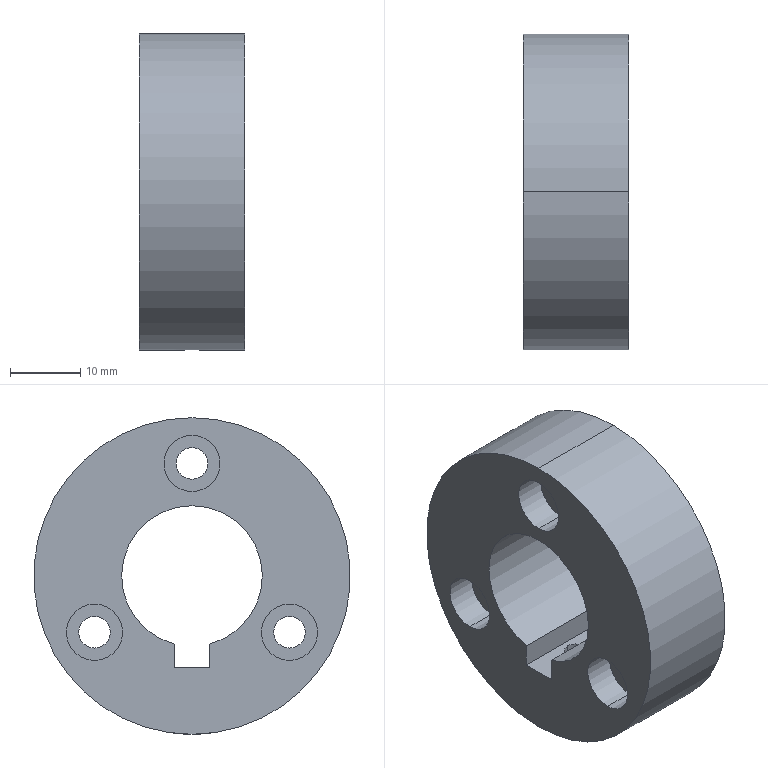Component | SolidWorks | 18-1 | 1 solid | 26 faces | box 15 x 45 x 45 mm | volume 17661 mm3 | cylinder 18 | plane 8 | commonest cylinder face diameters 8 x6 4.5 x6 3.3 x2 20 x2 45 x2
build123d program:
from build123d import *

# Parameters (mm, degrees)
SKETCH1_R                                       = 22.5
SKETCH1_R_2                                     = 10
EXTRUDE1_DEPTH                                  = 15
SKETCH2_W                                       = 5
SKETCH2_H                                       = 5
EXTRUDE2_DEPTH                                  = 36.178
M4_HEX_SOCKET_HEAD_CAP_SCREW_CBORE1_D           = 4.5
M4_HEX_SOCKET_HEAD_CAP_SCREW_CBORE1_CBORE_D     = 8
M4_HEX_SOCKET_HEAD_CAP_SCREW_CBORE1_CBORE_DEPTH = 4.4
M4_TAPPED_HOLE1_D                               = 3.3
M4_TAPPED_HOLE1_DEPTH                           = 9.5


with BuildPart() as part:
    # Sketch1 → Extrude1 (new body)
    with BuildSketch(Plane(origin=(0, 0, 0), x_dir=(1, 0, 0), z_dir=(0, 1, 0))):
        with Locations(Location((0, 0, 0), (0, 0, 270))):
            Circle(SKETCH1_R)
        with Locations(Location((0, 0, 0), (0, 0, 270))):
            Circle(SKETCH1_R_2, mode=Mode.SUBTRACT)
    extrude(amount=EXTRUDE1_DEPTH)

    # Sketch2 → Extrude2 (cut, through all)
    with BuildSketch(Plane(origin=(0, 15, 0), x_dir=(1, 0, 0), z_dir=(0, 1, 0))):
        with Locations((0, -10.5)):
            Rectangle(SKETCH2_W, SKETCH2_H)
    extrude(amount=-EXTRUDE2_DEPTH, mode=Mode.SUBTRACT)

    # M4 Hex Socket Head Cap Screw CBORE1 (through all)
    with Locations(Plane(origin=(13.856, 0, 8), x_dir=(0, 0, -1), z_dir=(0, -1, 0))):
        with Locations((0, 0), (0, -27.713), (24, -13.856)):
            CounterBoreHole(M4_HEX_SOCKET_HEAD_CAP_SCREW_CBORE1_D / 2, M4_HEX_SOCKET_HEAD_CAP_SCREW_CBORE1_CBORE_D / 2, M4_HEX_SOCKET_HEAD_CAP_SCREW_CBORE1_CBORE_DEPTH)

    # M4 Tapped Hole1
    with Locations(Plane(origin=(0, 0, 13), x_dir=(-1, 0, 0), z_dir=(0, 0, -1))):
        with Locations((0, 7.5)):
            Hole(M4_TAPPED_HOLE1_D / 2, depth=M4_TAPPED_HOLE1_DEPTH)


solid = part.part

# Placed as in the assembly
solid = solid.moved(Location((63.5, -32.5, 30), (180, 0, -90)))
STEP:
#1=CARTESIAN_POINT('',(2.795,-1.215,0.2977));
#2=VERTEX_POINT('',#1);
#3=CARTESIAN_POINT('',(2.73,-1.28,0.2953));
#4=VERTEX_POINT('',#3);
#5=CARTESIAN_POINT('',(2.795,-1.215,0.2977));
#6=CARTESIAN_POINT('',(2.787,-1.215,0.2977));
#7=CARTESIAN_POINT('',(2.778,-1.216,0.2975));
#8=CARTESIAN_POINT('',(2.766,-1.221,0.2972));
#9=CARTESIAN_POINT('',(2.763,-1.223,0.2971));
#10=CARTESIAN_POINT('',(2.756,-1.228,0.2968));
#11=CARTESIAN_POINT('',(2.752,-1.231,0.2966));
#12=CARTESIAN_POINT('',(2.743,-1.24,0.2962));
#13=CARTESIAN_POINT('',(2.739,-1.247,0.2958));
#14=CARTESIAN_POINT('',(2.732,-1.262,0.2954));
#15=CARTESIAN_POINT('',(2.73,-1.271,0.2953));
#16=CARTESIAN_POINT('',(2.73,-1.28,0.2953));
#17=B_SPLINE_CURVE_WITH_KNOTS('',3,(#5,#6,#7,#8,#9,#10,#11,#12,#13,#14,#15,#16),.UNSPECIFIED.,.F.,.F.,(4,2,2,2,2,4),(0.007741,0.008386,0.008708,0.00903,0.009675,0.01032),.UNSPECIFIED.);
#18=EDGE_CURVE('',#2,#4,#17,.T.);
#19=ORIENTED_EDGE('',*,*,#18,.F.);
#20=CARTESIAN_POINT('',(2.795,-1.215,0.6693));
#21=VERTEX_POINT('',#20);
#22=CARTESIAN_POINT('',(2.795,-1.215,0.6693));
#23=DIRECTION('',(0.,0.,1.));
#24=VECTOR('',#23,39.37);
#25=LINE('',#22,#24);
#26=EDGE_CURVE('',#2,#21,#25,.T.);
#27=ORIENTED_EDGE('',*,*,#26,.T.);
#28=CARTESIAN_POINT('',(2.795,-1.344,0.6693));
#29=VERTEX_POINT('',#28);
#30=CARTESIAN_POINT('',(2.795,-1.28,0.6693));
#31=DIRECTION('',(0.,0.,1.));
#32=DIRECTION('',(0.,-1.,0.));
#33=AXIS2_PLACEMENT_3D('',#30,#31,#32);
#34=CIRCLE('',#33,0.06496);
#35=EDGE_CURVE('',#21,#29,#34,.T.);
#36=ORIENTED_EDGE('',*,*,#35,.T.);
#37=CARTESIAN_POINT('',(2.795,-1.344,0.2977));
#38=VERTEX_POINT('',#37);
#39=CARTESIAN_POINT('',(2.795,-1.344,0.6693));
#40=DIRECTION('',(0.,0.,1.));
#41=VECTOR('',#40,39.37);
#42=LINE('',#39,#41);
#43=EDGE_CURVE('',#38,#29,#42,.T.);
#44=ORIENTED_EDGE('',*,*,#43,.F.);
#45=CARTESIAN_POINT('',(2.73,-1.28,0.2953));
#46=CARTESIAN_POINT('',(2.73,-1.284,0.2953));
#47=CARTESIAN_POINT('',(2.731,-1.288,0.2953));
#48=CARTESIAN_POINT('',(2.732,-1.296,0.2954));
#49=CARTESIAN_POINT('',(2.734,-1.3,0.2955));
#50=CARTESIAN_POINT('',(2.737,-1.308,0.2957));
#51=CARTESIAN_POINT('',(2.739,-1.312,0.2959));
#52=CARTESIAN_POINT('',(2.744,-1.319,0.2962));
#53=CARTESIAN_POINT('',(2.746,-1.322,0.2963));
#54=CARTESIAN_POINT('',(2.755,-1.331,0.2968));
#55=CARTESIAN_POINT('',(2.763,-1.336,0.2971));
#56=CARTESIAN_POINT('',(2.778,-1.343,0.2975));
#57=CARTESIAN_POINT('',(2.787,-1.344,0.2977));
#58=CARTESIAN_POINT('',(2.795,-1.344,0.2977));
#59=B_SPLINE_CURVE_WITH_KNOTS('',3,(#45,#46,#47,#48,#49,#50,#51,#52,#53,#54,#55,#56,#57,#58),.UNSPECIFIED.,.F.,.F.,(4,2,2,2,2,2,4),(0.,0.0003226,0.0006452,0.0009678,0.00129,0.001936,0.002581),.UNSPECIFIED.);
#60=EDGE_CURVE('',#4,#38,#59,.T.);
#61=ORIENTED_EDGE('',*,*,#60,.F.);
#62=EDGE_LOOP('',(#19,#27,#36,#44,#61));
#63=FACE_OUTER_BOUND('',#62,.T.);
#64=CARTESIAN_POINT('',(2.795,-1.28,0.6693));
#65=DIRECTION('',(0.,0.,1.));
#66=DIRECTION('',(0.,-1.,0.));
#67=AXIS2_PLACEMENT_3D('',#64,#65,#66);
#68=CYLINDRICAL_SURFACE('',#67,0.06496);
#69=ADVANCED_FACE('',(#63),#68,.F.);
#70=CARTESIAN_POINT('',(2.673,-0.734,0.7087));
#71=VERTEX_POINT('',#70);
#72=CARTESIAN_POINT('',(2.673,-0.734,1.024));
#73=VERTEX_POINT('',#72);
#74=CARTESIAN_POINT('',(2.673,-0.734,0.8661));
#75=DIRECTION('',(-1.,-0.,0.));
#76=DIRECTION('',(0.,0.,1.));
#77=AXIS2_PLACEMENT_3D('',#74,#75,#76);
#78=CIRCLE('',#77,0.1575);
#79=EDGE_CURVE('',#71,#73,#78,.T.);
#80=ORIENTED_EDGE('',*,*,#79,.F.);
#81=CARTESIAN_POINT('',(2.5,-0.734,0.7087));
#82=VERTEX_POINT('',#81);
#83=CARTESIAN_POINT('',(2.5,-0.734,0.7087));
#84=DIRECTION('',(-1.,-0.,0.));
#85=VECTOR('',#84,39.37);
#86=LINE('',#83,#85);
#87=EDGE_CURVE('',#71,#82,#86,.T.);
#88=ORIENTED_EDGE('',*,*,#87,.T.);
#89=CARTESIAN_POINT('',(2.5,-0.734,1.024));
#90=VERTEX_POINT('',#89);
#91=CARTESIAN_POINT('',(2.5,-0.734,0.8661));
#92=DIRECTION('',(-1.,-0.,0.));
#93=DIRECTION('',(0.,0.,1.));
#94=AXIS2_PLACEMENT_3D('',#91,#92,#93);
#95=CIRCLE('',#94,0.1575);
#96=EDGE_CURVE('',#82,#90,#95,.T.);
#97=ORIENTED_EDGE('',*,*,#96,.T.);
#98=CARTESIAN_POINT('',(2.5,-0.734,1.024));
#99=DIRECTION('',(-1.,-0.,0.));
#100=VECTOR('',#99,39.37);
#101=LINE('',#98,#100);
#102=EDGE_CURVE('',#73,#90,#101,.T.);
#103=ORIENTED_EDGE('',*,*,#102,.F.);
#104=EDGE_LOOP('',(#80,#88,#97,#103));
#105=FACE_OUTER_BOUND('',#104,.T.);
#106=CARTESIAN_POINT('',(2.5,-0.734,0.8661));
#107=DIRECTION('',(-1.,-0.,0.));
#108=DIRECTION('',(0.,0.,1.));
#109=AXIS2_PLACEMENT_3D('',#106,#107,#108);
#110=CYLINDRICAL_SURFACE('',#109,0.1575);
#111=ADVANCED_FACE('',(#105),#110,.F.);
#112=CARTESIAN_POINT('',(3.091,-0.734,0.7776));
#113=VERTEX_POINT('',#112);
#114=CARTESIAN_POINT('',(3.091,-0.734,0.9547));
#115=VERTEX_POINT('',#114);
#116=CARTESIAN_POINT('',(3.091,-0.734,0.8661));
#117=DIRECTION('',(-1.,-0.,0.));
#118=DIRECTION('',(0.,0.,1.));
#119=AXIS2_PLACEMENT_3D('',#116,#117,#118);
#120=CIRCLE('',#119,0.08858);
#121=EDGE_CURVE('',#113,#115,#120,.T.);
#122=ORIENTED_EDGE('',*,*,#121,.F.);
#123=CARTESIAN_POINT('',(2.673,-0.734,0.7776));
#124=VERTEX_POINT('',#123);
#125=CARTESIAN_POINT('',(2.5,-0.734,0.7776));
#126=DIRECTION('',(-1.,-0.,0.));
#127=VECTOR('',#126,39.37);
#128=LINE('',#125,#127);
#129=EDGE_CURVE('',#113,#124,#128,.T.);
#130=ORIENTED_EDGE('',*,*,#129,.T.);
#131=CARTESIAN_POINT('',(2.673,-0.734,0.9547));
#132=VERTEX_POINT('',#131);
#133=CARTESIAN_POINT('',(2.673,-0.734,0.8661));
#134=DIRECTION('',(-1.,-0.,0.));
#135=DIRECTION('',(0.,0.,1.));
#136=AXIS2_PLACEMENT_3D('',#133,#134,#135);
#137=CIRCLE('',#136,0.08858);
#138=EDGE_CURVE('',#124,#132,#137,.T.);
#139=ORIENTED_EDGE('',*,*,#138,.T.);
#140=CARTESIAN_POINT('',(2.5,-0.734,0.9547));
#141=DIRECTION('',(-1.,-0.,0.));
#142=VECTOR('',#141,39.37);
#143=LINE('',#140,#142);
#144=EDGE_CURVE('',#115,#132,#143,.T.);
#145=ORIENTED_EDGE('',*,*,#144,.F.);
#146=EDGE_LOOP('',(#122,#130,#139,#145));
#147=FACE_OUTER_BOUND('',#146,.T.);
#148=CARTESIAN_POINT('',(2.5,-0.734,0.8661));
#149=DIRECTION('',(-1.,-0.,0.));
#150=DIRECTION('',(0.,0.,1.));
#151=AXIS2_PLACEMENT_3D('',#148,#149,#150);
#152=CYLINDRICAL_SURFACE('',#151,0.08858);
#153=ADVANCED_FACE('',(#147),#152,.F.);
#154=CARTESIAN_POINT('',(2.673,-1.825,0.7087));
#155=VERTEX_POINT('',#154);
#156=CARTESIAN_POINT('',(2.673,-1.825,1.024));
#157=VERTEX_POINT('',#156);
#158=CARTESIAN_POINT('',(2.673,-1.825,0.8661));
#159=DIRECTION('',(-1.,-0.,0.));
#160=DIRECTION('',(0.,0.,1.));
#161=AXIS2_PLACEMENT_3D('',#158,#159,#160);
#162=CIRCLE('',#161,0.1575);
#163=EDGE_CURVE('',#155,#157,#162,.T.);
#164=ORIENTED_EDGE('',*,*,#163,.F.);
#165=CARTESIAN_POINT('',(2.5,-1.825,0.7087));
#166=VERTEX_POINT('',#165);
#167=CARTESIAN_POINT('',(2.5,-1.825,0.7087));
#168=DIRECTION('',(-1.,-0.,0.));
#169=VECTOR('',#168,39.37);
#170=LINE('',#167,#169);
#171=EDGE_CURVE('',#155,#166,#170,.T.);
#172=ORIENTED_EDGE('',*,*,#171,.T.);
#173=CARTESIAN_POINT('',(2.5,-1.825,1.024));
#174=VERTEX_POINT('',#173);
#175=CARTESIAN_POINT('',(2.5,-1.825,0.8661));
#176=DIRECTION('',(-1.,-0.,0.));
#177=DIRECTION('',(0.,0.,1.));
#178=AXIS2_PLACEMENT_3D('',#175,#176,#177);
#179=CIRCLE('',#178,0.1575);
#180=EDGE_CURVE('',#166,#174,#179,.T.);
#181=ORIENTED_EDGE('',*,*,#180,.T.);
#182=CARTESIAN_POINT('',(2.5,-1.825,1.024));
#183=DIRECTION('',(-1.,-0.,0.));
#184=VECTOR('',#183,39.37);
#185=LINE('',#182,#184);
#186=EDGE_CURVE('',#157,#174,#185,.T.);
#187=ORIENTED_EDGE('',*,*,#186,.F.);
#188=EDGE_LOOP('',(#164,#172,#181,#187));
#189=FACE_OUTER_BOUND('',#188,.T.);
#190=CARTESIAN_POINT('',(2.5,-1.825,0.8661));
#191=DIRECTION('',(-1.,-0.,0.));
#192=DIRECTION('',(0.,0.,1.));
#193=AXIS2_PLACEMENT_3D('',#190,#191,#192);
#194=CYLINDRICAL_SURFACE('',#193,0.1575);
#195=ADVANCED_FACE('',(#189),#194,.F.);
#196=CARTESIAN_POINT('',(3.091,-1.825,0.7776));
#197=VERTEX_POINT('',#196);
#198=CARTESIAN_POINT('',(3.091,-1.825,0.9547));
#199=VERTEX_POINT('',#198);
#200=CARTESIAN_POINT('',(3.091,-1.825,0.8661));
#201=DIRECTION('',(-1.,-0.,0.));
#202=DIRECTION('',(0.,0.,1.));
#203=AXIS2_PLACEMENT_3D('',#200,#201,#202);
#204=CIRCLE('',#203,0.08858);
#205=EDGE_CURVE('',#197,#199,#204,.T.);
#206=ORIENTED_EDGE('',*,*,#205,.F.);
#207=CARTESIAN_POINT('',(2.673,-1.825,0.7776));
#208=VERTEX_POINT('',#207);
#209=CARTESIAN_POINT('',(2.5,-1.825,0.7776));
#210=DIRECTION('',(-1.,-0.,0.));
#211=VECTOR('',#210,39.37);
#212=LINE('',#209,#211);
#213=EDGE_CURVE('',#197,#208,#212,.T.);
#214=ORIENTED_EDGE('',*,*,#213,.T.);
#215=CARTESIAN_POINT('',(2.673,-1.825,0.9547));
#216=VERTEX_POINT('',#215);
#217=CARTESIAN_POINT('',(2.673,-1.825,0.8661));
#218=DIRECTION('',(-1.,-0.,0.));
#219=DIRECTION('',(0.,0.,1.));
#220=AXIS2_PLACEMENT_3D('',#217,#218,#219);
#221=CIRCLE('',#220,0.08858);
#222=EDGE_CURVE('',#208,#216,#221,.T.);
#223=ORIENTED_EDGE('',*,*,#222,.T.);
#224=CARTESIAN_POINT('',(2.5,-1.825,0.9547));
#225=DIRECTION('',(-1.,-0.,0.));
#226=VECTOR('',#225,39.37);
#227=LINE('',#224,#226);
#228=EDGE_CURVE('',#199,#216,#227,.T.);
#229=ORIENTED_EDGE('',*,*,#228,.F.);
#230=EDGE_LOOP('',(#206,#214,#223,#229));
#231=FACE_OUTER_BOUND('',#230,.T.);
#232=CARTESIAN_POINT('',(2.5,-1.825,0.8661));
#233=DIRECTION('',(-1.,-0.,0.));
#234=DIRECTION('',(0.,0.,1.));
#235=AXIS2_PLACEMENT_3D('',#232,#233,#234);
#236=CYLINDRICAL_SURFACE('',#235,0.08858);
#237=ADVANCED_FACE('',(#231),#236,.F.);
#238=CARTESIAN_POINT('',(2.673,-1.28,1.654));
#239=VERTEX_POINT('',#238);
#240=CARTESIAN_POINT('',(2.673,-1.28,1.969));
#241=VERTEX_POINT('',#240);
#242=CARTESIAN_POINT('',(2.673,-1.28,1.811));
#243=DIRECTION('',(-1.,-0.,0.));
#244=DIRECTION('',(0.,0.,1.));
#245=AXIS2_PLACEMENT_3D('',#242,#243,#244);
#246=CIRCLE('',#245,0.1575);
#247=EDGE_CURVE('',#239,#241,#246,.T.);
#248=ORIENTED_EDGE('',*,*,#247,.F.);
#249=CARTESIAN_POINT('',(2.5,-1.28,1.654));
#250=VERTEX_POINT('',#249);
#251=CARTESIAN_POINT('',(2.5,-1.28,1.654));
#252=DIRECTION('',(-1.,-0.,0.));
#253=VECTOR('',#252,39.37);
#254=LINE('',#251,#253);
#255=EDGE_CURVE('',#239,#250,#254,.T.);
#256=ORIENTED_EDGE('',*,*,#255,.T.);
#257=CARTESIAN_POINT('',(2.5,-1.28,1.969));
#258=VERTEX_POINT('',#257);
#259=CARTESIAN_POINT('',(2.5,-1.28,1.811));
#260=DIRECTION('',(-1.,-0.,0.));
#261=DIRECTION('',(0.,0.,1.));
#262=AXIS2_PLACEMENT_3D('',#259,#260,#261);
#263=CIRCLE('',#262,0.1575);
#264=EDGE_CURVE('',#250,#258,#263,.T.);
#265=ORIENTED_EDGE('',*,*,#264,.T.);
#266=CARTESIAN_POINT('',(2.5,-1.28,1.969));
#267=DIRECTION('',(-1.,-0.,0.));
#268=VECTOR('',#267,39.37);
#269=LINE('',#266,#268);
#270=EDGE_CURVE('',#241,#258,#269,.T.);
#271=ORIENTED_EDGE('',*,*,#270,.F.);
#272=EDGE_LOOP('',(#248,#256,#265,#271));
#273=FACE_OUTER_BOUND('',#272,.T.);
#274=CARTESIAN_POINT('',(2.5,-1.28,1.811));
#275=DIRECTION('',(-1.,-0.,0.));
#276=DIRECTION('',(0.,0.,1.));
#277=AXIS2_PLACEMENT_3D('',#274,#275,#276);
#278=CYLINDRICAL_SURFACE('',#277,0.1575);
#279=ADVANCED_FACE('',(#273),#278,.F.);
#280=CARTESIAN_POINT('',(3.091,-1.28,1.722));
#281=VERTEX_POINT('',#280);
#282=CARTESIAN_POINT('',(3.091,-1.28,1.9));
#283=VERTEX_POINT('',#282);
#284=CARTESIAN_POINT('',(3.091,-1.28,1.811));
#285=DIRECTION('',(-1.,-0.,0.));
#286=DIRECTION('',(0.,0.,1.));
#287=AXIS2_PLACEMENT_3D('',#284,#285,#286);
#288=CIRCLE('',#287,0.08858);
#289=EDGE_CURVE('',#281,#283,#288,.T.);
#290=ORIENTED_EDGE('',*,*,#289,.F.);
#291=CARTESIAN_POINT('',(2.673,-1.28,1.722));
#292=VERTEX_POINT('',#291);
#293=CARTESIAN_POINT('',(2.5,-1.28,1.722));
#294=DIRECTION('',(-1.,-0.,0.));
#295=VECTOR('',#294,39.37);
#296=LINE('',#293,#295);
#297=EDGE_CURVE('',#281,#292,#296,.T.);
#298=ORIENTED_EDGE('',*,*,#297,.T.);
#299=CARTESIAN_POINT('',(2.673,-1.28,1.9));
#300=VERTEX_POINT('',#299);
#301=CARTESIAN_POINT('',(2.673,-1.28,1.811));
#302=DIRECTION('',(-1.,-0.,0.));
#303=DIRECTION('',(0.,0.,1.));
#304=AXIS2_PLACEMENT_3D('',#301,#302,#303);
#305=CIRCLE('',#304,0.08858);
#306=EDGE_CURVE('',#292,#300,#305,.T.);
#307=ORIENTED_EDGE('',*,*,#306,.T.);
#308=CARTESIAN_POINT('',(2.5,-1.28,1.9));
#309=DIRECTION('',(-1.,-0.,0.));
#310=VECTOR('',#309,39.37);
#311=LINE('',#308,#310);
#312=EDGE_CURVE('',#283,#300,#311,.T.);
#313=ORIENTED_EDGE('',*,*,#312,.F.);
#314=EDGE_LOOP('',(#290,#298,#307,#313));
#315=FACE_OUTER_BOUND('',#314,.T.);
#316=CARTESIAN_POINT('',(2.5,-1.28,1.811));
#317=DIRECTION('',(-1.,-0.,0.));
#318=DIRECTION('',(0.,0.,1.));
#319=AXIS2_PLACEMENT_3D('',#316,#317,#318);
#320=CYLINDRICAL_SURFACE('',#319,0.08858);
#321=ADVANCED_FACE('',(#315),#320,.F.);
#322=CARTESIAN_POINT('',(3.091,-1.181,0.7999));
#323=VERTEX_POINT('',#322);
#324=CARTESIAN_POINT('',(3.091,-1.28,1.575));
#325=VERTEX_POINT('',#324);
#326=CARTESIAN_POINT('',(3.091,-1.28,1.181));
#327=DIRECTION('',(1.,0.,-0.));
#328=DIRECTION('',(0.,-0.,-1.));
#329=AXIS2_PLACEMENT_3D('',#326,#327,#328);
#330=CIRCLE('',#329,0.3937);
#331=EDGE_CURVE('',#323,#325,#330,.T.);
#332=ORIENTED_EDGE('',*,*,#331,.T.);
#333=CARTESIAN_POINT('',(2.5,-1.28,1.575));
#334=VERTEX_POINT('',#333);
#335=CARTESIAN_POINT('',(3.091,-1.28,1.575));
#336=DIRECTION('',(-1.,-0.,0.));
#337=VECTOR('',#336,39.37);
#338=LINE('',#335,#337);
#339=EDGE_CURVE('',#325,#334,#338,.T.);
#340=ORIENTED_EDGE('',*,*,#339,.T.);
#341=CARTESIAN_POINT('',(2.5,-1.181,0.7999));
#342=VERTEX_POINT('',#341);
#343=CARTESIAN_POINT('',(2.5,-1.28,1.181));
#344=DIRECTION('',(1.,0.,-0.));
#345=DIRECTION('',(0.,-0.,-1.));
#346=AXIS2_PLACEMENT_3D('',#343,#344,#345);
#347=CIRCLE('',#346,0.3937);
#348=EDGE_CURVE('',#342,#334,#347,.T.);
#349=ORIENTED_EDGE('',*,*,#348,.F.);
#350=CARTESIAN_POINT('',(3.091,-1.181,0.7999));
#351=DIRECTION('',(-1.,-0.,0.));
#352=VECTOR('',#351,39.37);
#353=LINE('',#350,#352);
#354=EDGE_CURVE('',#323,#342,#353,.T.);
#355=ORIENTED_EDGE('',*,*,#354,.F.);
#356=EDGE_LOOP('',(#332,#340,#349,#355));
#357=FACE_OUTER_BOUND('',#356,.T.);
#358=CARTESIAN_POINT('',(3.091,-1.28,1.181));
#359=DIRECTION('',(-1.,-0.,0.));
#360=DIRECTION('',(0.,0.,1.));
#361=AXIS2_PLACEMENT_3D('',#358,#359,#360);
#362=CYLINDRICAL_SURFACE('',#361,0.3937);
#363=ADVANCED_FACE('',(#357),#362,.F.);
#364=CARTESIAN_POINT('',(3.091,-1.28,0.2953));
#365=VERTEX_POINT('',#364);
#366=CARTESIAN_POINT('',(3.091,-1.28,2.067));
#367=VERTEX_POINT('',#366);
#368=CARTESIAN_POINT('',(3.091,-1.28,1.181));
#369=DIRECTION('',(1.,0.,-0.));
#370=DIRECTION('',(0.,-0.,-1.));
#371=AXIS2_PLACEMENT_3D('',#368,#369,#370);
#372=CIRCLE('',#371,0.8858);
#373=EDGE_CURVE('',#365,#367,#372,.T.);
#374=ORIENTED_EDGE('',*,*,#373,.F.);
#375=CARTESIAN_POINT('',(2.86,-1.28,0.2953));
#376=VERTEX_POINT('',#375);
#377=CARTESIAN_POINT('',(3.091,-1.28,0.2953));
#378=DIRECTION('',(-1.,-0.,0.));
#379=VECTOR('',#378,39.37);
#380=LINE('',#377,#379);
#381=EDGE_CURVE('',#365,#376,#380,.T.);
#382=ORIENTED_EDGE('',*,*,#381,.T.);
#383=CARTESIAN_POINT('',(2.86,-1.28,0.2953));
#384=CARTESIAN_POINT('',(2.86,-1.271,0.2953));
#385=CARTESIAN_POINT('',(2.859,-1.262,0.2954));
#386=CARTESIAN_POINT('',(2.852,-1.247,0.2958));
#387=CARTESIAN_POINT('',(2.847,-1.24,0.2962));
#388=CARTESIAN_POINT('',(2.838,-1.231,0.2966));
#389=CARTESIAN_POINT('',(2.835,-1.228,0.2968));
#390=CARTESIAN_POINT('',(2.828,-1.223,0.2971));
#391=CARTESIAN_POINT('',(2.824,-1.221,0.2972));
#392=CARTESIAN_POINT('',(2.816,-1.218,0.2974));
#393=CARTESIAN_POINT('',(2.812,-1.217,0.2975));
#394=CARTESIAN_POINT('',(2.804,-1.215,0.2976));
#395=CARTESIAN_POINT('',(2.8,-1.215,0.2977));
#396=CARTESIAN_POINT('',(2.795,-1.215,0.2977));
#397=B_SPLINE_CURVE_WITH_KNOTS('',3,(#383,#384,#385,#386,#387,#388,#389,#390,#391,#392,#393,#394,#395,#396),.UNSPECIFIED.,.F.,.F.,(4,2,2,2,2,2,4),(0.00516,0.005806,0.006451,0.006773,0.007096,0.007419,0.007741),.UNSPECIFIED.);
#398=EDGE_CURVE('',#376,#2,#397,.T.);
#399=ORIENTED_EDGE('',*,*,#398,.T.);
#400=ORIENTED_EDGE('',*,*,#18,.T.);
#401=CARTESIAN_POINT('',(2.5,-1.28,0.2953));
#402=VERTEX_POINT('',#401);
#403=CARTESIAN_POINT('',(3.091,-1.28,0.2953));
#404=DIRECTION('',(-1.,-0.,0.));
#405=VECTOR('',#404,39.37);
#406=LINE('',#403,#405);
#407=EDGE_CURVE('',#4,#402,#406,.T.);
#408=ORIENTED_EDGE('',*,*,#407,.T.);
#409=CARTESIAN_POINT('',(2.5,-1.28,2.067));
#410=VERTEX_POINT('',#409);
#411=CARTESIAN_POINT('',(2.5,-1.28,1.181));
#412=DIRECTION('',(1.,0.,-0.));
#413=DIRECTION('',(0.,-0.,-1.));
#414=AXIS2_PLACEMENT_3D('',#411,#412,#413);
#415=CIRCLE('',#414,0.8858);
#416=EDGE_CURVE('',#402,#410,#415,.T.);
#417=ORIENTED_EDGE('',*,*,#416,.T.);
#418=CARTESIAN_POINT('',(3.091,-1.28,2.067));
#419=DIRECTION('',(-1.,-0.,0.));
#420=VECTOR('',#419,39.37);
#421=LINE('',#418,#420);
#422=EDGE_CURVE('',#367,#410,#421,.T.);
#423=ORIENTED_EDGE('',*,*,#422,.F.);
#424=EDGE_LOOP('',(#374,#382,#399,#400,#408,#417,#423));
#425=FACE_OUTER_BOUND('',#424,.T.);
#426=CARTESIAN_POINT('',(3.091,-1.28,1.181));
#427=DIRECTION('',(-1.,-0.,0.));
#428=DIRECTION('',(0.,0.,1.));
#429=AXIS2_PLACEMENT_3D('',#426,#427,#428);
#430=CYLINDRICAL_SURFACE('',#429,0.8858);
#431=ADVANCED_FACE('',(#425),#430,.T.);
#432=CARTESIAN_POINT('',(2.5,-0.734,0.8661));
#433=DIRECTION('',(-1.,-0.,0.));
#434=DIRECTION('',(0.,0.,1.));
#435=AXIS2_PLACEMENT_3D('',#432,#433,#434);
#436=CIRCLE('',#435,0.1575);
#437=EDGE_CURVE('',#90,#82,#436,.T.);
#438=ORIENTED_EDGE('',*,*,#437,.F.);
#439=ORIENTED_EDGE('',*,*,#96,.F.);
#440=EDGE_LOOP('',(#438,#439));
#441=FACE_BOUND('',#440,.T.);
#442=CARTESIAN_POINT('',(2.5,-1.825,0.8661));
#443=DIRECTION('',(-1.,-0.,0.));
#444=DIRECTION('',(0.,0.,1.));
#445=AXIS2_PLACEMENT_3D('',#442,#443,#444);
#446=CIRCLE('',#445,0.1575);
#447=EDGE_CURVE('',#174,#166,#446,.T.);
#448=ORIENTED_EDGE('',*,*,#447,.F.);
#449=ORIENTED_EDGE('',*,*,#180,.F.);
#450=EDGE_LOOP('',(#448,#449));
#451=FACE_BOUND('',#450,.T.);
#452=CARTESIAN_POINT('',(2.5,-1.28,1.181));
#453=DIRECTION('',(1.,0.,-0.));
#454=DIRECTION('',(0.,-0.,-1.));
#455=AXIS2_PLACEMENT_3D('',#452,#453,#454);
#456=CIRCLE('',#455,0.8858);
#457=EDGE_CURVE('',#410,#402,#456,.T.);
#458=ORIENTED_EDGE('',*,*,#457,.F.);
#459=ORIENTED_EDGE('',*,*,#416,.F.);
#460=EDGE_LOOP('',(#458,#459));
#461=FACE_OUTER_BOUND('',#460,.T.);
#462=ORIENTED_EDGE('',*,*,#348,.T.);
#463=CARTESIAN_POINT('',(2.5,-1.378,0.7999));
#464=VERTEX_POINT('',#463);
#465=CARTESIAN_POINT('',(2.5,-1.28,1.181));
#466=DIRECTION('',(1.,0.,-0.));
#467=DIRECTION('',(0.,-0.,-1.));
#468=AXIS2_PLACEMENT_3D('',#465,#466,#467);
#469=CIRCLE('',#468,0.3937);
#470=EDGE_CURVE('',#334,#464,#469,.T.);
#471=ORIENTED_EDGE('',*,*,#470,.T.);
#472=CARTESIAN_POINT('',(2.5,-1.378,0.6693));
#473=VERTEX_POINT('',#472);
#474=CARTESIAN_POINT('',(2.5,-1.378,0.8661));
#475=DIRECTION('',(-0.,-0.,-1.));
#476=VECTOR('',#475,39.37);
#477=LINE('',#474,#476);
#478=EDGE_CURVE('',#464,#473,#477,.T.);
#479=ORIENTED_EDGE('',*,*,#478,.T.);
#480=CARTESIAN_POINT('',(2.5,-1.181,0.6693));
#481=VERTEX_POINT('',#480);
#482=CARTESIAN_POINT('',(2.5,-1.378,0.6693));
#483=DIRECTION('',(-0.,1.,-0.));
#484=VECTOR('',#483,39.37);
#485=LINE('',#482,#484);
#486=EDGE_CURVE('',#473,#481,#485,.T.);
#487=ORIENTED_EDGE('',*,*,#486,.T.);
#488=CARTESIAN_POINT('',(2.5,-1.181,0.8661));
#489=DIRECTION('',(0.,0.,1.));
#490=VECTOR('',#489,39.37);
#491=LINE('',#488,#490);
#492=EDGE_CURVE('',#481,#342,#491,.T.);
#493=ORIENTED_EDGE('',*,*,#492,.T.);
#494=EDGE_LOOP('',(#462,#471,#479,#487,#493));
#495=FACE_BOUND('',#494,.T.);
#496=CARTESIAN_POINT('',(2.5,-1.28,1.811));
#497=DIRECTION('',(-1.,-0.,0.));
#498=DIRECTION('',(0.,0.,1.));
#499=AXIS2_PLACEMENT_3D('',#496,#497,#498);
#500=CIRCLE('',#499,0.1575);
#501=EDGE_CURVE('',#258,#250,#500,.T.);
#502=ORIENTED_EDGE('',*,*,#501,.F.);
#503=ORIENTED_EDGE('',*,*,#264,.F.);
#504=EDGE_LOOP('',(#502,#503));
#505=FACE_BOUND('',#504,.T.);
#506=CARTESIAN_POINT('',(2.5,-1.28,1.181));
#507=DIRECTION('',(1.,0.,-0.));
#508=DIRECTION('',(-0.,-0.,-1.));
#509=AXIS2_PLACEMENT_3D('',#506,#507,#508);
#510=PLANE('',#509);
#511=ADVANCED_FACE('',(#441,#451,#461,#495,#505),#510,.F.);
#512=CARTESIAN_POINT('',(3.091,-0.734,0.8661));
#513=DIRECTION('',(-1.,-0.,0.));
#514=DIRECTION('',(0.,0.,1.));
#515=AXIS2_PLACEMENT_3D('',#512,#513,#514);
#516=CIRCLE('',#515,0.08858);
#517=EDGE_CURVE('',#115,#113,#516,.T.);
#518=ORIENTED_EDGE('',*,*,#517,.T.);
#519=ORIENTED_EDGE('',*,*,#121,.T.);
#520=EDGE_LOOP('',(#518,#519));
#521=FACE_BOUND('',#520,.T.);
#522=CARTESIAN_POINT('',(3.091,-1.825,0.8661));
#523=DIRECTION('',(-1.,-0.,0.));
#524=DIRECTION('',(0.,0.,1.));
#525=AXIS2_PLACEMENT_3D('',#522,#523,#524);
#526=CIRCLE('',#525,0.08858);
#527=EDGE_CURVE('',#199,#197,#526,.T.);
#528=ORIENTED_EDGE('',*,*,#527,.T.);
#529=ORIENTED_EDGE('',*,*,#205,.T.);
#530=EDGE_LOOP('',(#528,#529));
#531=FACE_BOUND('',#530,.T.);
#532=CARTESIAN_POINT('',(3.091,-1.28,1.811));
#533=DIRECTION('',(-1.,-0.,0.));
#534=DIRECTION('',(0.,0.,1.));
#535=AXIS2_PLACEMENT_3D('',#532,#533,#534);
#536=CIRCLE('',#535,0.08858);
#537=EDGE_CURVE('',#283,#281,#536,.T.);
#538=ORIENTED_EDGE('',*,*,#537,.T.);
#539=ORIENTED_EDGE('',*,*,#289,.T.);
#540=EDGE_LOOP('',(#538,#539));
#541=FACE_BOUND('',#540,.T.);
#542=CARTESIAN_POINT('',(3.091,-1.378,0.7999));
#543=VERTEX_POINT('',#542);
#544=CARTESIAN_POINT('',(3.091,-1.378,0.6693));
#545=VERTEX_POINT('',#544);
#546=CARTESIAN_POINT('',(3.091,-1.378,0.8661));
#547=DIRECTION('',(-0.,-0.,-1.));
#548=VECTOR('',#547,39.37);
#549=LINE('',#546,#548);
#550=EDGE_CURVE('',#543,#545,#549,.T.);
#551=ORIENTED_EDGE('',*,*,#550,.F.);
#552=CARTESIAN_POINT('',(3.091,-1.28,1.181));
#553=DIRECTION('',(1.,0.,-0.));
#554=DIRECTION('',(0.,-0.,-1.));
#555=AXIS2_PLACEMENT_3D('',#552,#553,#554);
#556=CIRCLE('',#555,0.3937);
#557=EDGE_CURVE('',#325,#543,#556,.T.);
#558=ORIENTED_EDGE('',*,*,#557,.F.);
#559=ORIENTED_EDGE('',*,*,#331,.F.);
#560=CARTESIAN_POINT('',(3.091,-1.181,0.6693));
#561=VERTEX_POINT('',#560);
#562=CARTESIAN_POINT('',(3.091,-1.181,0.8661));
#563=DIRECTION('',(0.,0.,1.));
#564=VECTOR('',#563,39.37);
#565=LINE('',#562,#564);
#566=EDGE_CURVE('',#561,#323,#565,.T.);
#567=ORIENTED_EDGE('',*,*,#566,.F.);
#568=CARTESIAN_POINT('',(3.091,-1.378,0.6693));
#569=DIRECTION('',(-0.,1.,-0.));
#570=VECTOR('',#569,39.37);
#571=LINE('',#568,#570);
#572=EDGE_CURVE('',#545,#561,#571,.T.);
#573=ORIENTED_EDGE('',*,*,#572,.F.);
#574=EDGE_LOOP('',(#551,#558,#559,#567,#573));
#575=FACE_BOUND('',#574,.T.);
#576=CARTESIAN_POINT('',(3.091,-1.28,1.181));
#577=DIRECTION('',(1.,0.,-0.));
#578=DIRECTION('',(0.,-0.,-1.));
#579=AXIS2_PLACEMENT_3D('',#576,#577,#578);
#580=CIRCLE('',#579,0.8858);
#581=EDGE_CURVE('',#367,#365,#580,.T.);
#582=ORIENTED_EDGE('',*,*,#581,.T.);
#583=ORIENTED_EDGE('',*,*,#373,.T.);
#584=EDGE_LOOP('',(#582,#583));
#585=FACE_OUTER_BOUND('',#584,.T.);
#586=CARTESIAN_POINT('',(3.091,-1.28,1.181));
#587=DIRECTION('',(1.,0.,-0.));
#588=DIRECTION('',(-0.,-0.,-1.));
#589=AXIS2_PLACEMENT_3D('',#586,#587,#588);
#590=PLANE('',#589);
#591=ADVANCED_FACE('',(#521,#531,#541,#575,#585),#590,.T.);
#592=ORIENTED_EDGE('',*,*,#381,.F.);
#593=ORIENTED_EDGE('',*,*,#581,.F.);
#594=ORIENTED_EDGE('',*,*,#422,.T.);
#595=ORIENTED_EDGE('',*,*,#457,.T.);
#596=ORIENTED_EDGE('',*,*,#407,.F.);
#597=ORIENTED_EDGE('',*,*,#60,.T.);
#598=CARTESIAN_POINT('',(2.795,-1.344,0.2977));
#599=CARTESIAN_POINT('',(2.8,-1.344,0.2977));
#600=CARTESIAN_POINT('',(2.804,-1.344,0.2976));
#601=CARTESIAN_POINT('',(2.812,-1.342,0.2975));
#602=CARTESIAN_POINT('',(2.816,-1.341,0.2974));
#603=CARTESIAN_POINT('',(2.824,-1.338,0.2972));
#604=CARTESIAN_POINT('',(2.828,-1.336,0.2971));
#605=CARTESIAN_POINT('',(2.835,-1.331,0.2968));
#606=CARTESIAN_POINT('',(2.838,-1.328,0.2966));
#607=CARTESIAN_POINT('',(2.844,-1.322,0.2963));
#608=CARTESIAN_POINT('',(2.847,-1.319,0.2962));
#609=CARTESIAN_POINT('',(2.852,-1.312,0.2959));
#610=CARTESIAN_POINT('',(2.854,-1.308,0.2957));
#611=CARTESIAN_POINT('',(2.857,-1.3,0.2955));
#612=CARTESIAN_POINT('',(2.858,-1.296,0.2954));
#613=CARTESIAN_POINT('',(2.86,-1.288,0.2953));
#614=CARTESIAN_POINT('',(2.86,-1.284,0.2953));
#615=CARTESIAN_POINT('',(2.86,-1.28,0.2953));
#616=B_SPLINE_CURVE_WITH_KNOTS('',3,(#598,#599,#600,#601,#602,#603,#604,#605,#606,#607,#608,#609,#610,#611,#612,#613,#614,#615),.UNSPECIFIED.,.F.,.F.,(4,2,2,2,2,2,2,2,4),(0.002581,0.002903,0.003226,0.003548,0.003871,0.004193,0.004515,0.004838,0.00516),.UNSPECIFIED.);
#617=EDGE_CURVE('',#38,#376,#616,.T.);
#618=ORIENTED_EDGE('',*,*,#617,.T.);
#619=EDGE_LOOP('',(#592,#593,#594,#595,#596,#597,#618));
#620=FACE_OUTER_BOUND('',#619,.T.);
#621=CARTESIAN_POINT('',(3.091,-1.28,1.181));
#622=DIRECTION('',(-1.,-0.,0.));
#623=DIRECTION('',(0.,0.,1.));
#624=AXIS2_PLACEMENT_3D('',#621,#622,#623);
#625=CYLINDRICAL_SURFACE('',#624,0.8858);
#626=ADVANCED_FACE('',(#620),#625,.T.);
#627=ORIENTED_EDGE('',*,*,#339,.F.);
#628=ORIENTED_EDGE('',*,*,#557,.T.);
#629=CARTESIAN_POINT('',(3.091,-1.378,0.7999));
#630=DIRECTION('',(1.,0.,-0.));
#631=VECTOR('',#630,39.37);
#632=LINE('',#629,#631);
#633=EDGE_CURVE('',#464,#543,#632,.T.);
#634=ORIENTED_EDGE('',*,*,#633,.F.);
#635=ORIENTED_EDGE('',*,*,#470,.F.);
#636=EDGE_LOOP('',(#627,#628,#634,#635));
#637=FACE_OUTER_BOUND('',#636,.T.);
#638=CARTESIAN_POINT('',(3.091,-1.28,1.181));
#639=DIRECTION('',(-1.,-0.,0.));
#640=DIRECTION('',(0.,0.,1.));
#641=AXIS2_PLACEMENT_3D('',#638,#639,#640);
#642=CYLINDRICAL_SURFACE('',#641,0.3937);
#643=ADVANCED_FACE('',(#637),#642,.F.);
#644=ORIENTED_EDGE('',*,*,#633,.T.);
#645=ORIENTED_EDGE('',*,*,#550,.T.);
#646=CARTESIAN_POINT('',(2.5,-1.378,0.6693));
#647=DIRECTION('',(1.,0.,-0.));
#648=VECTOR('',#647,39.37);
#649=LINE('',#646,#648);
#650=EDGE_CURVE('',#473,#545,#649,.T.);
#651=ORIENTED_EDGE('',*,*,#650,.F.);
#652=ORIENTED_EDGE('',*,*,#478,.F.);
#653=EDGE_LOOP('',(#644,#645,#651,#652));
#654=FACE_OUTER_BOUND('',#653,.T.);
#655=CARTESIAN_POINT('',(2.5,-1.378,0.8661));
#656=DIRECTION('',(0.,-1.,0.));
#657=DIRECTION('',(-0.,-0.,-1.));
#658=AXIS2_PLACEMENT_3D('',#655,#656,#657);
#659=PLANE('',#658);
#660=ADVANCED_FACE('',(#654),#659,.F.);
#661=ORIENTED_EDGE('',*,*,#354,.T.);
#662=ORIENTED_EDGE('',*,*,#492,.F.);
#663=CARTESIAN_POINT('',(2.5,-1.181,0.6693));
#664=DIRECTION('',(1.,0.,-0.));
#665=VECTOR('',#664,39.37);
#666=LINE('',#663,#665);
#667=EDGE_CURVE('',#481,#561,#666,.T.);
#668=ORIENTED_EDGE('',*,*,#667,.T.);
#669=ORIENTED_EDGE('',*,*,#566,.T.);
#670=EDGE_LOOP('',(#661,#662,#668,#669));
#671=FACE_OUTER_BOUND('',#670,.T.);
#672=CARTESIAN_POINT('',(2.5,-1.181,0.8661));
#673=DIRECTION('',(-0.,1.,-0.));
#674=DIRECTION('',(0.,0.,1.));
#675=AXIS2_PLACEMENT_3D('',#672,#673,#674);
#676=PLANE('',#675);
#677=ADVANCED_FACE('',(#671),#676,.F.);
#678=CARTESIAN_POINT('',(2.795,-1.28,0.6693));
#679=DIRECTION('',(0.,0.,1.));
#680=DIRECTION('',(0.,-1.,0.));
#681=AXIS2_PLACEMENT_3D('',#678,#679,#680);
#682=CIRCLE('',#681,0.06496);
#683=EDGE_CURVE('',#29,#21,#682,.T.);
#684=ORIENTED_EDGE('',*,*,#683,.F.);
#685=ORIENTED_EDGE('',*,*,#35,.F.);
#686=EDGE_LOOP('',(#684,#685));
#687=FACE_BOUND('',#686,.T.);
#688=ORIENTED_EDGE('',*,*,#572,.T.);
#689=ORIENTED_EDGE('',*,*,#667,.F.);
#690=ORIENTED_EDGE('',*,*,#486,.F.);
#691=ORIENTED_EDGE('',*,*,#650,.T.);
#692=EDGE_LOOP('',(#688,#689,#690,#691));
#693=FACE_OUTER_BOUND('',#692,.T.);
#694=CARTESIAN_POINT('',(2.5,-1.378,0.6693));
#695=DIRECTION('',(-0.,-0.,-1.));
#696=DIRECTION('',(-0.,1.,-0.));
#697=AXIS2_PLACEMENT_3D('',#694,#695,#696);
#698=PLANE('',#697);
#699=ADVANCED_FACE('',(#687,#693),#698,.F.);
#700=ORIENTED_EDGE('',*,*,#297,.F.);
#701=ORIENTED_EDGE('',*,*,#537,.F.);
#702=ORIENTED_EDGE('',*,*,#312,.T.);
#703=CARTESIAN_POINT('',(2.673,-1.28,1.811));
#704=DIRECTION('',(-1.,-0.,0.));
#705=DIRECTION('',(0.,0.,1.));
#706=AXIS2_PLACEMENT_3D('',#703,#704,#705);
#707=CIRCLE('',#706,0.08858);
#708=EDGE_CURVE('',#300,#292,#707,.T.);
#709=ORIENTED_EDGE('',*,*,#708,.T.);
#710=EDGE_LOOP('',(#700,#701,#702,#709));
#711=FACE_OUTER_BOUND('',#710,.T.);
#712=CARTESIAN_POINT('',(2.5,-1.28,1.811));
#713=DIRECTION('',(-1.,-0.,0.));
#714=DIRECTION('',(0.,0.,1.));
#715=AXIS2_PLACEMENT_3D('',#712,#713,#714);
#716=CYLINDRICAL_SURFACE('',#715,0.08858);
#717=ADVANCED_FACE('',(#711),#716,.F.);
#718=ORIENTED_EDGE('',*,*,#708,.F.);
#719=ORIENTED_EDGE('',*,*,#306,.F.);
#720=EDGE_LOOP('',(#718,#719));
#721=FACE_BOUND('',#720,.T.);
#722=CARTESIAN_POINT('',(2.673,-1.28,1.811));
#723=DIRECTION('',(-1.,-0.,0.));
#724=DIRECTION('',(0.,0.,1.));
#725=AXIS2_PLACEMENT_3D('',#722,#723,#724);
#726=CIRCLE('',#725,0.1575);
#727=EDGE_CURVE('',#241,#239,#726,.T.);
#728=ORIENTED_EDGE('',*,*,#727,.T.);
#729=ORIENTED_EDGE('',*,*,#247,.T.);
#730=EDGE_LOOP('',(#728,#729));
#731=FACE_OUTER_BOUND('',#730,.T.);
#732=CARTESIAN_POINT('',(2.673,-1.191,1.811));
#733=DIRECTION('',(1.,0.,-0.));
#734=DIRECTION('',(-0.,-0.,-1.));
#735=AXIS2_PLACEMENT_3D('',#732,#733,#734);
#736=PLANE('',#735);
#737=ADVANCED_FACE('',(#721,#731),#736,.F.);
#738=ORIENTED_EDGE('',*,*,#255,.F.);
#739=ORIENTED_EDGE('',*,*,#727,.F.);
#740=ORIENTED_EDGE('',*,*,#270,.T.);
#741=ORIENTED_EDGE('',*,*,#501,.T.);
#742=EDGE_LOOP('',(#738,#739,#740,#741));
#743=FACE_OUTER_BOUND('',#742,.T.);
#744=CARTESIAN_POINT('',(2.5,-1.28,1.811));
#745=DIRECTION('',(-1.,-0.,0.));
#746=DIRECTION('',(0.,0.,1.));
#747=AXIS2_PLACEMENT_3D('',#744,#745,#746);
#748=CYLINDRICAL_SURFACE('',#747,0.1575);
#749=ADVANCED_FACE('',(#743),#748,.F.);
#750=ORIENTED_EDGE('',*,*,#213,.F.);
#751=ORIENTED_EDGE('',*,*,#527,.F.);
#752=ORIENTED_EDGE('',*,*,#228,.T.);
#753=CARTESIAN_POINT('',(2.673,-1.825,0.8661));
#754=DIRECTION('',(-1.,-0.,0.));
#755=DIRECTION('',(0.,0.,1.));
#756=AXIS2_PLACEMENT_3D('',#753,#754,#755);
#757=CIRCLE('',#756,0.08858);
#758=EDGE_CURVE('',#216,#208,#757,.T.);
#759=ORIENTED_EDGE('',*,*,#758,.T.);
#760=EDGE_LOOP('',(#750,#751,#752,#759));
#761=FACE_OUTER_BOUND('',#760,.T.);
#762=CARTESIAN_POINT('',(2.5,-1.825,0.8661));
#763=DIRECTION('',(-1.,-0.,0.));
#764=DIRECTION('',(0.,0.,1.));
#765=AXIS2_PLACEMENT_3D('',#762,#763,#764);
#766=CYLINDRICAL_SURFACE('',#765,0.08858);
#767=ADVANCED_FACE('',(#761),#766,.F.);
#768=ORIENTED_EDGE('',*,*,#758,.F.);
#769=ORIENTED_EDGE('',*,*,#222,.F.);
#770=EDGE_LOOP('',(#768,#769));
#771=FACE_BOUND('',#770,.T.);
#772=CARTESIAN_POINT('',(2.673,-1.825,0.8661));
#773=DIRECTION('',(-1.,-0.,0.));
#774=DIRECTION('',(0.,0.,1.));
#775=AXIS2_PLACEMENT_3D('',#772,#773,#774);
#776=CIRCLE('',#775,0.1575);
#777=EDGE_CURVE('',#157,#155,#776,.T.);
#778=ORIENTED_EDGE('',*,*,#777,.T.);
#779=ORIENTED_EDGE('',*,*,#163,.T.);
#780=EDGE_LOOP('',(#778,#779));
#781=FACE_OUTER_BOUND('',#780,.T.);
#782=CARTESIAN_POINT('',(2.673,-1.736,0.8661));
#783=DIRECTION('',(1.,0.,-0.));
#784=DIRECTION('',(-0.,-0.,-1.));
#785=AXIS2_PLACEMENT_3D('',#782,#783,#784);
#786=PLANE('',#785);
#787=ADVANCED_FACE('',(#771,#781),#786,.F.);
#788=ORIENTED_EDGE('',*,*,#171,.F.);
#789=ORIENTED_EDGE('',*,*,#777,.F.);
#790=ORIENTED_EDGE('',*,*,#186,.T.);
#791=ORIENTED_EDGE('',*,*,#447,.T.);
#792=EDGE_LOOP('',(#788,#789,#790,#791));
#793=FACE_OUTER_BOUND('',#792,.T.);
#794=CARTESIAN_POINT('',(2.5,-1.825,0.8661));
#795=DIRECTION('',(-1.,-0.,0.));
#796=DIRECTION('',(0.,0.,1.));
#797=AXIS2_PLACEMENT_3D('',#794,#795,#796);
#798=CYLINDRICAL_SURFACE('',#797,0.1575);
#799=ADVANCED_FACE('',(#793),#798,.F.);
#800=ORIENTED_EDGE('',*,*,#129,.F.);
#801=ORIENTED_EDGE('',*,*,#517,.F.);
#802=ORIENTED_EDGE('',*,*,#144,.T.);
#803=CARTESIAN_POINT('',(2.673,-0.734,0.8661));
#804=DIRECTION('',(-1.,-0.,0.));
#805=DIRECTION('',(0.,0.,1.));
#806=AXIS2_PLACEMENT_3D('',#803,#804,#805);
#807=CIRCLE('',#806,0.08858);
#808=EDGE_CURVE('',#132,#124,#807,.T.);
#809=ORIENTED_EDGE('',*,*,#808,.T.);
#810=EDGE_LOOP('',(#800,#801,#802,#809));
#811=FACE_OUTER_BOUND('',#810,.T.);
#812=CARTESIAN_POINT('',(2.5,-0.734,0.8661));
#813=DIRECTION('',(-1.,-0.,0.));
#814=DIRECTION('',(0.,0.,1.));
#815=AXIS2_PLACEMENT_3D('',#812,#813,#814);
#816=CYLINDRICAL_SURFACE('',#815,0.08858);
#817=ADVANCED_FACE('',(#811),#816,.F.);
#818=ORIENTED_EDGE('',*,*,#808,.F.);
#819=ORIENTED_EDGE('',*,*,#138,.F.);
#820=EDGE_LOOP('',(#818,#819));
#821=FACE_BOUND('',#820,.T.);
#822=CARTESIAN_POINT('',(2.673,-0.734,0.8661));
#823=DIRECTION('',(-1.,-0.,0.));
#824=DIRECTION('',(0.,0.,1.));
#825=AXIS2_PLACEMENT_3D('',#822,#823,#824);
#826=CIRCLE('',#825,0.1575);
#827=EDGE_CURVE('',#73,#71,#826,.T.);
#828=ORIENTED_EDGE('',*,*,#827,.T.);
#829=ORIENTED_EDGE('',*,*,#79,.T.);
#830=EDGE_LOOP('',(#828,#829));
#831=FACE_OUTER_BOUND('',#830,.T.);
#832=CARTESIAN_POINT('',(2.673,-0.6454,0.8661));
#833=DIRECTION('',(1.,0.,-0.));
#834=DIRECTION('',(-0.,-0.,-1.));
#835=AXIS2_PLACEMENT_3D('',#832,#833,#834);
#836=PLANE('',#835);
#837=ADVANCED_FACE('',(#821,#831),#836,.F.);
#838=ORIENTED_EDGE('',*,*,#87,.F.);
#839=ORIENTED_EDGE('',*,*,#827,.F.);
#840=ORIENTED_EDGE('',*,*,#102,.T.);
#841=ORIENTED_EDGE('',*,*,#437,.T.);
#842=EDGE_LOOP('',(#838,#839,#840,#841));
#843=FACE_OUTER_BOUND('',#842,.T.);
#844=CARTESIAN_POINT('',(2.5,-0.734,0.8661));
#845=DIRECTION('',(-1.,-0.,0.));
#846=DIRECTION('',(0.,0.,1.));
#847=AXIS2_PLACEMENT_3D('',#844,#845,#846);
#848=CYLINDRICAL_SURFACE('',#847,0.1575);
#849=ADVANCED_FACE('',(#843),#848,.F.);
#850=ORIENTED_EDGE('',*,*,#26,.F.);
#851=ORIENTED_EDGE('',*,*,#398,.F.);
#852=ORIENTED_EDGE('',*,*,#617,.F.);
#853=ORIENTED_EDGE('',*,*,#43,.T.);
#854=ORIENTED_EDGE('',*,*,#683,.T.);
#855=EDGE_LOOP('',(#850,#851,#852,#853,#854));
#856=FACE_OUTER_BOUND('',#855,.T.);
#857=CARTESIAN_POINT('',(2.795,-1.28,0.6693));
#858=DIRECTION('',(0.,0.,1.));
#859=DIRECTION('',(0.,-1.,0.));
#860=AXIS2_PLACEMENT_3D('',#857,#858,#859);
#861=CYLINDRICAL_SURFACE('',#860,0.06496);
#862=ADVANCED_FACE('',(#856),#861,.F.);
#863=CLOSED_SHELL('',(#69,#111,#153,#195,#237,#279,#321,#363,#431,#511,#591,#626,#643,#660,#677,#699,#717,#737,#749,#767,#787,#799,#817,#837,#849,#862));
#864=MANIFOLD_SOLID_BREP('',#863);
#865=CARTESIAN_POINT('',(0.,0.,0.));
#866=DIRECTION('',(0.,0.,1.));
#867=DIRECTION('',(1.,0.,0.));
#868=AXIS2_PLACEMENT_3D('',#865,#866,#867);
#869=(LENGTH_UNIT()NAMED_UNIT(*)SI_UNIT($,.METRE.));
#870=LENGTH_MEASURE_WITH_UNIT(LENGTH_MEASURE(0.0254),#869);
#871=DIMENSIONAL_EXPONENTS(1.,0.,0.,0.,0.,0.,0.);
#872=(CONVERSION_BASED_UNIT('',#870)LENGTH_UNIT()NAMED_UNIT(#871));
#873=UNCERTAINTY_MEASURE_WITH_UNIT(LENGTH_MEASURE(0.00001),#872,'','');
#874=(NAMED_UNIT(*)PLANE_ANGLE_UNIT()SI_UNIT($,.RADIAN.));
#875=(NAMED_UNIT(*)SI_UNIT($,.STERADIAN.)SOLID_ANGLE_UNIT());
#876=(GEOMETRIC_REPRESENTATION_CONTEXT(3)GLOBAL_UNCERTAINTY_ASSIGNED_CONTEXT((#873))GLOBAL_UNIT_ASSIGNED_CONTEXT((#872,#874,#875))REPRESENTATION_CONTEXT('',''));
#877=ADVANCED_BREP_SHAPE_REPRESENTATION('',(#864,#868),#876);
#878=COLOUR_RGB('',0.7922,0.8196,0.9333);
#879=FILL_AREA_STYLE_COLOUR('',#878);
#880=FILL_AREA_STYLE('',(#879));
#881=SURFACE_STYLE_FILL_AREA(#880);
#882=SURFACE_SIDE_STYLE('',(#881));
#883=SURFACE_STYLE_USAGE(.BOTH.,#882);
#884=PRESENTATION_STYLE_ASSIGNMENT((#883));
#885=STYLED_ITEM('',(#884),#864);
#886=(LENGTH_UNIT()NAMED_UNIT(*)SI_UNIT($,.METRE.));
#887=LENGTH_MEASURE_WITH_UNIT(LENGTH_MEASURE(0.0254),#886);
#888=DIMENSIONAL_EXPONENTS(1.,0.,0.,0.,0.,0.,0.);
#889=(CONVERSION_BASED_UNIT('',#887)LENGTH_UNIT()NAMED_UNIT(#888));
#890=UNCERTAINTY_MEASURE_WITH_UNIT(LENGTH_MEASURE(0.00001),#889,'','');
#891=(NAMED_UNIT(*)PLANE_ANGLE_UNIT()SI_UNIT($,.RADIAN.));
#892=(NAMED_UNIT(*)SI_UNIT($,.STERADIAN.)SOLID_ANGLE_UNIT());
#893=(GEOMETRIC_REPRESENTATION_CONTEXT(3)GLOBAL_UNCERTAINTY_ASSIGNED_CONTEXT((#890))GLOBAL_UNIT_ASSIGNED_CONTEXT((#889,#891,#892))REPRESENTATION_CONTEXT('',''));
#894=MECHANICAL_DESIGN_GEOMETRIC_PRESENTATION_REPRESENTATION('',(#885),#893);
#895=PRESENTATION_LAYER_ASSIGNMENT('','',(#885));